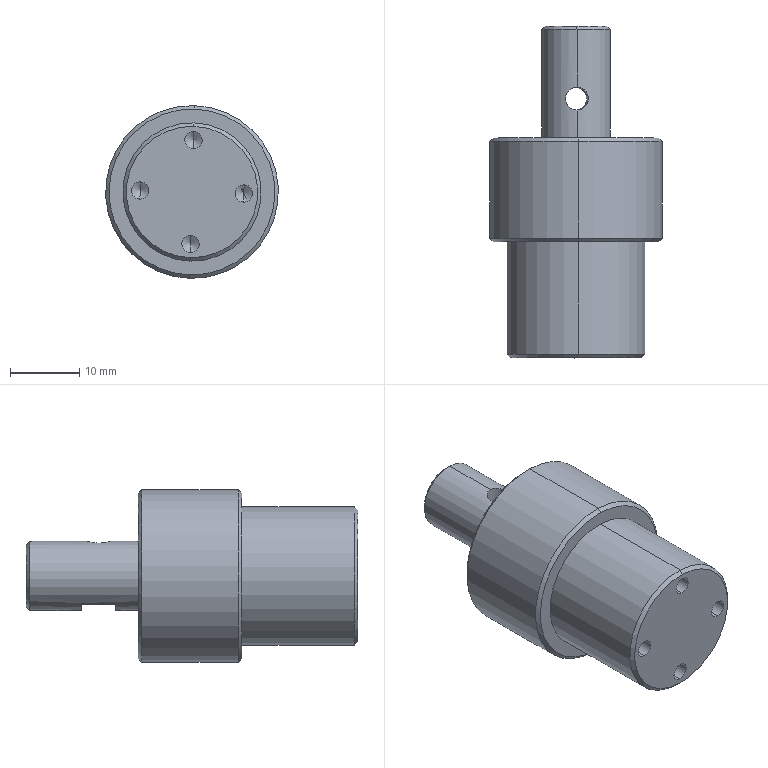Component | SolidWorks | H2020022-0415-1-1 | 1 solid | 43 faces | volume 13556 mm3 | cylinder 18 | cone 18 | plane 7 | commonest cylinder face diameters 2.5 x8 3.3 x4 20 x2 25 x2 10 x2 | material 45#Steel